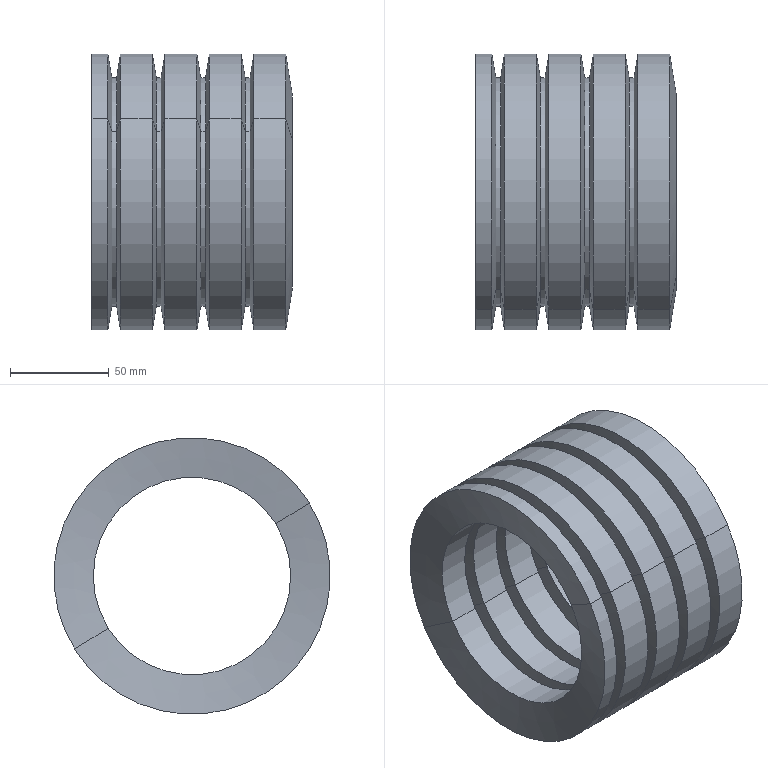Component | SolidWorks | DiscSpring-1 | 1 solid | 72 faces | box 101.37 x 140 x 140 mm | volume 580259 mm3 | cone 36 | cylinder 36 | commonest cylinder face diameters 140 x10 100 x10 116 x8 124 x8
build123d program:
from build123d import *

# Parameters (mm, degrees)
LPATTERN1_COUNT = 4
LPATTERN1_PITCH = 22.523


with BuildPart() as part:
    # Sketch1 → Revolve1 (revolve)
    with BuildSketch(Plane.XY, mode=Mode.PRIVATE) as revolve1_sk:
        Polygon((50, -11.267), (50, -3.168), (62, -1.267), (62, 1.267), (50, 3.168), (50, 11.267), (50, 19.367), (70, 22.535), (70, 14.435), (58, 12.534), (58, 10), (70, 8.1), (70, -8.1), align=None)
    revolve1 = revolve(revolve1_sk.sketch.rotate(Axis((0, 0, 0), (0, 1, 0)), 90), axis=Axis((0, 0, 0), (0, 1, 0)))

    # LPattern1: Revolve1 ×4
    with Locations(*[(0, i * LPATTERN1_PITCH, 0) for i in range(1, LPATTERN1_COUNT)]):
        add(revolve1)


solid = part.part

# Placed as in the assembly
solid = solid.moved(Location((-157.396, 0, 0), (0, 0, 90)))